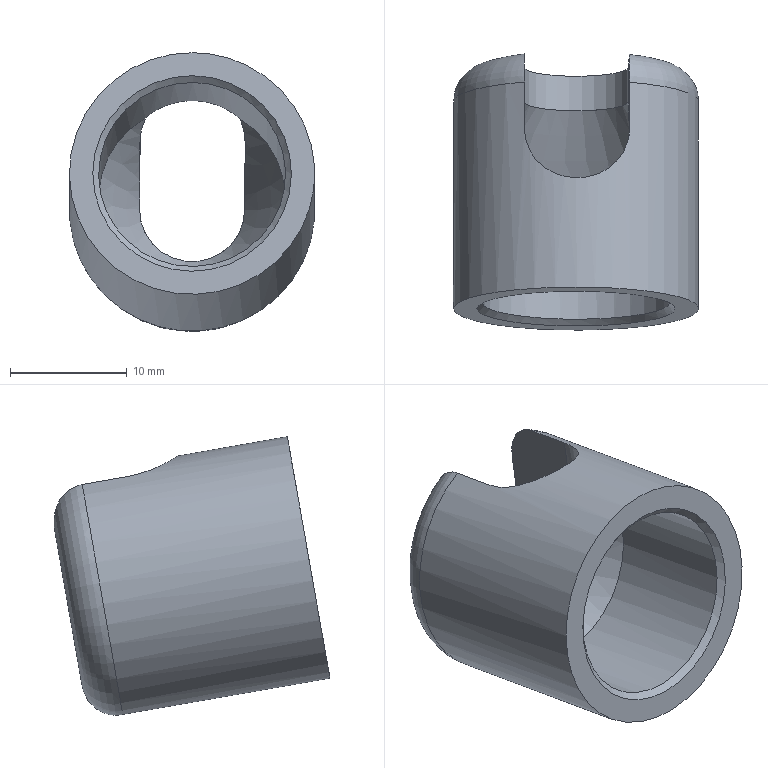Component | NX | BALL_JOINT_OUTER_SLEEVE | 1 solid | 14 faces | volume 3348 mm3 | plane 7 | cylinder 4 | cone 2 | torus 1 | commonest cylinder face diameters 9 x2 21 x1 16 x1